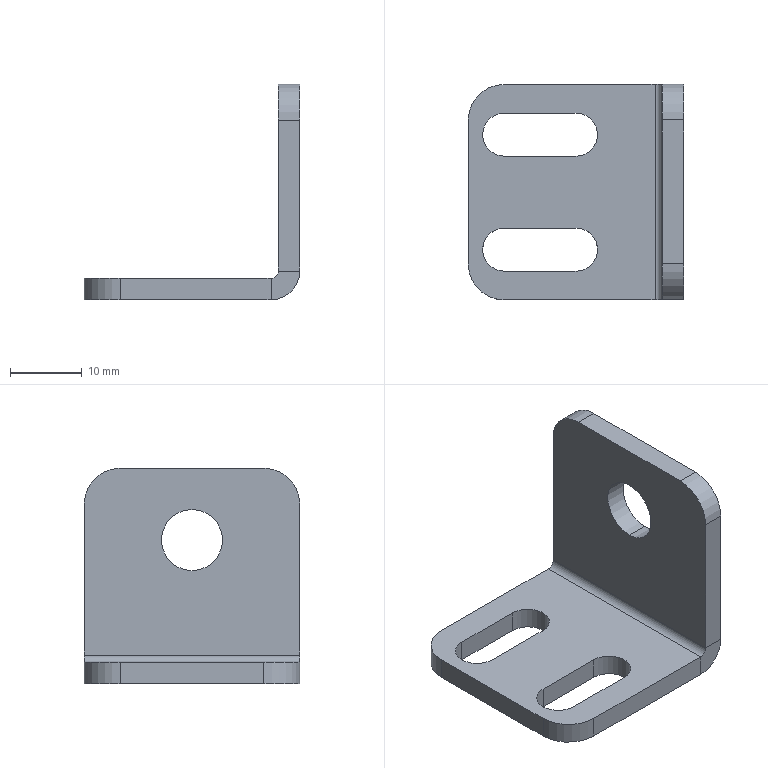Component | SolidWorks | GuideWheelAssembly3-1_RollerBracket1-1 | 1 solid | 28 faces | box 30 x 30 x 30 mm | volume 4269 mm3 | plane 16 | cylinder 12 | commonest cylinder face diameters 6 x4 10 x4 8.5 x2 2 x1 8 x1
STEP:
#1=CARTESIAN_POINT('',(-20.078,-9.252,1.014));
#2=VERTEX_POINT('',#1);
#3=CARTESIAN_POINT('',(-20.078,-9.252,1.348));
#4=VERTEX_POINT('',#3);
#5=CARTESIAN_POINT('',(-20.078,-9.252,1.181));
#6=DIRECTION('',(-1.,-0.,0.));
#7=DIRECTION('',(0.,0.,1.));
#8=AXIS2_PLACEMENT_3D('',#5,#6,#7);
#9=CIRCLE('',#8,0.1673);
#10=EDGE_CURVE('',#2,#4,#9,.T.);
#11=ORIENTED_EDGE('',*,*,#10,.F.);
#12=CARTESIAN_POINT('',(-20.196,-9.252,1.014));
#13=VERTEX_POINT('',#12);
#14=CARTESIAN_POINT('',(-20.078,-9.252,1.014));
#15=DIRECTION('',(-1.,-0.,0.));
#16=VECTOR('',#15,39.37);
#17=LINE('',#14,#16);
#18=EDGE_CURVE('',#2,#13,#17,.T.);
#19=ORIENTED_EDGE('',*,*,#18,.T.);
#20=CARTESIAN_POINT('',(-20.196,-9.252,1.348));
#21=VERTEX_POINT('',#20);
#22=CARTESIAN_POINT('',(-20.196,-9.252,1.181));
#23=DIRECTION('',(-1.,-0.,0.));
#24=DIRECTION('',(0.,0.,1.));
#25=AXIS2_PLACEMENT_3D('',#22,#23,#24);
#26=CIRCLE('',#25,0.1673);
#27=EDGE_CURVE('',#13,#21,#26,.T.);
#28=ORIENTED_EDGE('',*,*,#27,.T.);
#29=CARTESIAN_POINT('',(-20.078,-9.252,1.348));
#30=DIRECTION('',(-1.,-0.,0.));
#31=VECTOR('',#30,39.37);
#32=LINE('',#29,#31);
#33=EDGE_CURVE('',#4,#21,#32,.T.);
#34=ORIENTED_EDGE('',*,*,#33,.F.);
#35=EDGE_LOOP('',(#11,#19,#28,#34));
#36=FACE_OUTER_BOUND('',#35,.T.);
#37=CARTESIAN_POINT('',(-20.078,-9.252,1.181));
#38=DIRECTION('',(-1.,-0.,0.));
#39=DIRECTION('',(0.,0.,1.));
#40=AXIS2_PLACEMENT_3D('',#37,#38,#39);
#41=CYLINDRICAL_SURFACE('',#40,0.1673);
#42=ADVANCED_FACE('',(#36),#41,.F.);
#43=CARTESIAN_POINT('',(-20.078,-8.661,0.5512));
#44=VERTEX_POINT('',#43);
#45=CARTESIAN_POINT('',(-20.196,-8.661,0.5512));
#46=VERTEX_POINT('',#45);
#47=CARTESIAN_POINT('',(-20.078,-8.661,0.5512));
#48=DIRECTION('',(-1.,-0.,0.));
#49=VECTOR('',#48,39.37);
#50=LINE('',#47,#49);
#51=EDGE_CURVE('',#44,#46,#50,.T.);
#52=ORIENTED_EDGE('',*,*,#51,.F.);
#53=CARTESIAN_POINT('',(-20.235,-8.661,0.3937));
#54=VERTEX_POINT('',#53);
#55=CARTESIAN_POINT('',(-20.235,-8.661,0.5512));
#56=DIRECTION('',(-0.,1.,-0.));
#57=DIRECTION('',(1.,0.,0.));
#58=AXIS2_PLACEMENT_3D('',#55,#56,#57);
#59=CIRCLE('',#58,0.1575);
#60=EDGE_CURVE('',#44,#54,#59,.T.);
#61=ORIENTED_EDGE('',*,*,#60,.T.);
#62=CARTESIAN_POINT('',(-20.235,-8.661,0.5118));
#63=VERTEX_POINT('',#62);
#64=CARTESIAN_POINT('',(-20.235,-8.661,0.5118));
#65=DIRECTION('',(-0.,-0.,-1.));
#66=VECTOR('',#65,39.37);
#67=LINE('',#64,#66);
#68=EDGE_CURVE('',#63,#54,#67,.T.);
#69=ORIENTED_EDGE('',*,*,#68,.F.);
#70=CARTESIAN_POINT('',(-20.235,-8.661,0.5512));
#71=DIRECTION('',(-0.,1.,-0.));
#72=DIRECTION('',(-1.,0.,0.));
#73=AXIS2_PLACEMENT_3D('',#70,#71,#72);
#74=CIRCLE('',#73,0.03937);
#75=EDGE_CURVE('',#46,#63,#74,.T.);
#76=ORIENTED_EDGE('',*,*,#75,.F.);
#77=EDGE_LOOP('',(#52,#61,#69,#76));
#78=FACE_OUTER_BOUND('',#77,.T.);
#79=CARTESIAN_POINT('',(-20.078,-8.661,0.5512));
#80=DIRECTION('',(-0.,1.,-0.));
#81=DIRECTION('',(-1.,-0.,0.));
#82=AXIS2_PLACEMENT_3D('',#79,#80,#81);
#83=PLANE('',#82);
#84=ADVANCED_FACE('',(#78),#83,.T.);
#85=CARTESIAN_POINT('',(-20.196,-8.661,1.378));
#86=VERTEX_POINT('',#85);
#87=CARTESIAN_POINT('',(-20.196,-8.661,1.575));
#88=DIRECTION('',(0.,-0.,-1.));
#89=VECTOR('',#88,39.37);
#90=LINE('',#87,#89);
#91=EDGE_CURVE('',#86,#46,#90,.T.);
#92=ORIENTED_EDGE('',*,*,#91,.F.);
#93=CARTESIAN_POINT('',(-20.078,-8.661,1.378));
#94=VERTEX_POINT('',#93);
#95=CARTESIAN_POINT('',(-20.235,-8.661,1.378));
#96=DIRECTION('',(1.,0.,-0.));
#97=VECTOR('',#96,39.37);
#98=LINE('',#95,#97);
#99=EDGE_CURVE('',#86,#94,#98,.T.);
#100=ORIENTED_EDGE('',*,*,#99,.T.);
#101=CARTESIAN_POINT('',(-20.078,-8.661,1.575));
#102=DIRECTION('',(0.,-0.,-1.));
#103=VECTOR('',#102,39.37);
#104=LINE('',#101,#103);
#105=EDGE_CURVE('',#94,#44,#104,.T.);
#106=ORIENTED_EDGE('',*,*,#105,.T.);
#107=ORIENTED_EDGE('',*,*,#51,.T.);
#108=EDGE_LOOP('',(#92,#100,#106,#107));
#109=FACE_OUTER_BOUND('',#108,.T.);
#110=CARTESIAN_POINT('',(-20.235,-8.661,0.5118));
#111=DIRECTION('',(-0.,1.,-0.));
#112=DIRECTION('',(-1.,-0.,0.));
#113=AXIS2_PLACEMENT_3D('',#110,#111,#112);
#114=PLANE('',#113);
#115=ADVANCED_FACE('',(#109),#114,.T.);
#116=CARTESIAN_POINT('',(-20.235,-9.843,0.3937));
#117=VERTEX_POINT('',#116);
#118=CARTESIAN_POINT('',(-20.235,-9.843,0.5118));
#119=VERTEX_POINT('',#118);
#120=CARTESIAN_POINT('',(-20.235,-9.843,0.3937));
#121=DIRECTION('',(0.,0.,1.));
#122=VECTOR('',#121,39.37);
#123=LINE('',#120,#122);
#124=EDGE_CURVE('',#117,#119,#123,.T.);
#125=ORIENTED_EDGE('',*,*,#124,.F.);
#126=CARTESIAN_POINT('',(-20.078,-9.843,0.5512));
#127=VERTEX_POINT('',#126);
#128=CARTESIAN_POINT('',(-20.235,-9.843,0.5512));
#129=DIRECTION('',(-0.,1.,-0.));
#130=DIRECTION('',(1.,0.,0.));
#131=AXIS2_PLACEMENT_3D('',#128,#129,#130);
#132=CIRCLE('',#131,0.1575);
#133=EDGE_CURVE('',#127,#117,#132,.T.);
#134=ORIENTED_EDGE('',*,*,#133,.F.);
#135=CARTESIAN_POINT('',(-20.196,-9.843,0.5512));
#136=VERTEX_POINT('',#135);
#137=CARTESIAN_POINT('',(-20.196,-9.843,0.5512));
#138=DIRECTION('',(1.,0.,-0.));
#139=VECTOR('',#138,39.37);
#140=LINE('',#137,#139);
#141=EDGE_CURVE('',#136,#127,#140,.T.);
#142=ORIENTED_EDGE('',*,*,#141,.F.);
#143=CARTESIAN_POINT('',(-20.235,-9.843,0.5512));
#144=DIRECTION('',(-0.,1.,-0.));
#145=DIRECTION('',(-1.,0.,0.));
#146=AXIS2_PLACEMENT_3D('',#143,#144,#145);
#147=CIRCLE('',#146,0.03937);
#148=EDGE_CURVE('',#136,#119,#147,.T.);
#149=ORIENTED_EDGE('',*,*,#148,.T.);
#150=EDGE_LOOP('',(#125,#134,#142,#149));
#151=FACE_OUTER_BOUND('',#150,.T.);
#152=CARTESIAN_POINT('',(-20.235,-9.843,0.3937));
#153=DIRECTION('',(0.,-1.,0.));
#154=DIRECTION('',(1.,0.,-0.));
#155=AXIS2_PLACEMENT_3D('',#152,#153,#154);
#156=PLANE('',#155);
#157=ADVANCED_FACE('',(#151),#156,.T.);
#158=CARTESIAN_POINT('',(-21.062,-9.843,0.5118));
#159=VERTEX_POINT('',#158);
#160=CARTESIAN_POINT('',(-20.078,-9.843,0.5118));
#161=DIRECTION('',(-1.,-0.,0.));
#162=VECTOR('',#161,39.37);
#163=LINE('',#160,#162);
#164=EDGE_CURVE('',#119,#159,#163,.T.);
#165=ORIENTED_EDGE('',*,*,#164,.T.);
#166=CARTESIAN_POINT('',(-21.062,-9.843,0.3937));
#167=VERTEX_POINT('',#166);
#168=CARTESIAN_POINT('',(-21.062,-9.843,0.5512));
#169=DIRECTION('',(-0.,-0.,-1.));
#170=VECTOR('',#169,39.37);
#171=LINE('',#168,#170);
#172=EDGE_CURVE('',#159,#167,#171,.T.);
#173=ORIENTED_EDGE('',*,*,#172,.T.);
#174=CARTESIAN_POINT('',(-20.078,-9.843,0.3937));
#175=DIRECTION('',(-1.,-0.,0.));
#176=VECTOR('',#175,39.37);
#177=LINE('',#174,#176);
#178=EDGE_CURVE('',#117,#167,#177,.T.);
#179=ORIENTED_EDGE('',*,*,#178,.F.);
#180=ORIENTED_EDGE('',*,*,#124,.T.);
#181=EDGE_LOOP('',(#165,#173,#179,#180));
#182=FACE_OUTER_BOUND('',#181,.T.);
#183=CARTESIAN_POINT('',(-20.196,-9.843,0.5512));
#184=DIRECTION('',(0.,-1.,0.));
#185=DIRECTION('',(1.,0.,-0.));
#186=AXIS2_PLACEMENT_3D('',#183,#184,#185);
#187=PLANE('',#186);
#188=ADVANCED_FACE('',(#182),#187,.T.);
#189=CARTESIAN_POINT('',(-21.062,-9.055,0.3937));
#190=VERTEX_POINT('',#189);
#191=CARTESIAN_POINT('',(-20.668,-9.055,0.3937));
#192=VERTEX_POINT('',#191);
#193=CARTESIAN_POINT('',(-20.668,-9.055,0.3937));
#194=DIRECTION('',(1.,0.,-0.));
#195=VECTOR('',#194,39.37);
#196=LINE('',#193,#195);
#197=EDGE_CURVE('',#190,#192,#196,.T.);
#198=ORIENTED_EDGE('',*,*,#197,.T.);
#199=CARTESIAN_POINT('',(-20.668,-8.819,0.3937));
#200=VERTEX_POINT('',#199);
#201=CARTESIAN_POINT('',(-20.668,-8.937,0.3937));
#202=DIRECTION('',(0.,0.,1.));
#203=DIRECTION('',(0.,-1.,0.));
#204=AXIS2_PLACEMENT_3D('',#201,#202,#203);
#205=CIRCLE('',#204,0.1181);
#206=EDGE_CURVE('',#192,#200,#205,.T.);
#207=ORIENTED_EDGE('',*,*,#206,.T.);
#208=CARTESIAN_POINT('',(-21.062,-8.819,0.3937));
#209=VERTEX_POINT('',#208);
#210=CARTESIAN_POINT('',(-20.668,-8.819,0.3937));
#211=DIRECTION('',(-1.,-0.,0.));
#212=VECTOR('',#211,39.37);
#213=LINE('',#210,#212);
#214=EDGE_CURVE('',#200,#209,#213,.T.);
#215=ORIENTED_EDGE('',*,*,#214,.T.);
#216=CARTESIAN_POINT('',(-21.062,-8.937,0.3937));
#217=DIRECTION('',(0.,0.,1.));
#218=DIRECTION('',(0.,-1.,0.));
#219=AXIS2_PLACEMENT_3D('',#216,#217,#218);
#220=CIRCLE('',#219,0.1181);
#221=EDGE_CURVE('',#209,#190,#220,.T.);
#222=ORIENTED_EDGE('',*,*,#221,.T.);
#223=EDGE_LOOP('',(#198,#207,#215,#222));
#224=FACE_BOUND('',#223,.T.);
#225=CARTESIAN_POINT('',(-21.062,-9.685,0.3937));
#226=VERTEX_POINT('',#225);
#227=CARTESIAN_POINT('',(-20.668,-9.685,0.3937));
#228=VERTEX_POINT('',#227);
#229=CARTESIAN_POINT('',(-20.668,-9.685,0.3937));
#230=DIRECTION('',(1.,0.,-0.));
#231=VECTOR('',#230,39.37);
#232=LINE('',#229,#231);
#233=EDGE_CURVE('',#226,#228,#232,.T.);
#234=ORIENTED_EDGE('',*,*,#233,.T.);
#235=CARTESIAN_POINT('',(-20.668,-9.449,0.3937));
#236=VERTEX_POINT('',#235);
#237=CARTESIAN_POINT('',(-20.668,-9.567,0.3937));
#238=DIRECTION('',(0.,0.,1.));
#239=DIRECTION('',(0.,1.,0.));
#240=AXIS2_PLACEMENT_3D('',#237,#238,#239);
#241=CIRCLE('',#240,0.1181);
#242=EDGE_CURVE('',#228,#236,#241,.T.);
#243=ORIENTED_EDGE('',*,*,#242,.T.);
#244=CARTESIAN_POINT('',(-21.062,-9.449,0.3937));
#245=VERTEX_POINT('',#244);
#246=CARTESIAN_POINT('',(-20.668,-9.449,0.3937));
#247=DIRECTION('',(-1.,-0.,0.));
#248=VECTOR('',#247,39.37);
#249=LINE('',#246,#248);
#250=EDGE_CURVE('',#236,#245,#249,.T.);
#251=ORIENTED_EDGE('',*,*,#250,.T.);
#252=CARTESIAN_POINT('',(-21.062,-9.567,0.3937));
#253=DIRECTION('',(0.,0.,1.));
#254=DIRECTION('',(0.,1.,0.));
#255=AXIS2_PLACEMENT_3D('',#252,#253,#254);
#256=CIRCLE('',#255,0.1181);
#257=EDGE_CURVE('',#245,#226,#256,.T.);
#258=ORIENTED_EDGE('',*,*,#257,.T.);
#259=EDGE_LOOP('',(#234,#243,#251,#258));
#260=FACE_BOUND('',#259,.T.);
#261=CARTESIAN_POINT('',(-21.259,-8.858,0.3937));
#262=VERTEX_POINT('',#261);
#263=CARTESIAN_POINT('',(-21.259,-9.646,0.3937));
#264=VERTEX_POINT('',#263);
#265=CARTESIAN_POINT('',(-21.259,-8.661,0.3937));
#266=DIRECTION('',(0.,-1.,0.));
#267=VECTOR('',#266,39.37);
#268=LINE('',#265,#267);
#269=EDGE_CURVE('',#262,#264,#268,.T.);
#270=ORIENTED_EDGE('',*,*,#269,.F.);
#271=CARTESIAN_POINT('',(-21.062,-8.661,0.3937));
#272=VERTEX_POINT('',#271);
#273=CARTESIAN_POINT('',(-21.062,-8.858,0.3937));
#274=DIRECTION('',(-0.,-0.,-1.));
#275=DIRECTION('',(0.,1.,0.));
#276=AXIS2_PLACEMENT_3D('',#273,#274,#275);
#277=CIRCLE('',#276,0.1969);
#278=EDGE_CURVE('',#262,#272,#277,.T.);
#279=ORIENTED_EDGE('',*,*,#278,.T.);
#280=CARTESIAN_POINT('',(-20.078,-8.661,0.3937));
#281=DIRECTION('',(-1.,-0.,0.));
#282=VECTOR('',#281,39.37);
#283=LINE('',#280,#282);
#284=EDGE_CURVE('',#54,#272,#283,.T.);
#285=ORIENTED_EDGE('',*,*,#284,.F.);
#286=CARTESIAN_POINT('',(-20.235,-8.661,0.3937));
#287=DIRECTION('',(0.,-1.,0.));
#288=VECTOR('',#287,39.37);
#289=LINE('',#286,#288);
#290=EDGE_CURVE('',#54,#117,#289,.T.);
#291=ORIENTED_EDGE('',*,*,#290,.T.);
#292=ORIENTED_EDGE('',*,*,#178,.T.);
#293=CARTESIAN_POINT('',(-21.062,-9.646,0.3937));
#294=DIRECTION('',(-0.,-0.,-1.));
#295=DIRECTION('',(0.,1.,0.));
#296=AXIS2_PLACEMENT_3D('',#293,#294,#295);
#297=CIRCLE('',#296,0.1969);
#298=EDGE_CURVE('',#167,#264,#297,.T.);
#299=ORIENTED_EDGE('',*,*,#298,.T.);
#300=EDGE_LOOP('',(#270,#279,#285,#291,#292,#299));
#301=FACE_OUTER_BOUND('',#300,.T.);
#302=CARTESIAN_POINT('',(-20.078,-8.661,0.3937));
#303=DIRECTION('',(0.,0.,1.));
#304=DIRECTION('',(-0.,1.,-0.));
#305=AXIS2_PLACEMENT_3D('',#302,#303,#304);
#306=PLANE('',#305);
#307=ADVANCED_FACE('',(#224,#260,#301),#306,.F.);
#308=CARTESIAN_POINT('',(-21.259,-8.858,0.5118));
#309=VERTEX_POINT('',#308);
#310=CARTESIAN_POINT('',(-21.259,-9.646,0.5118));
#311=VERTEX_POINT('',#310);
#312=CARTESIAN_POINT('',(-21.259,-8.661,0.5118));
#313=DIRECTION('',(0.,-1.,0.));
#314=VECTOR('',#313,39.37);
#315=LINE('',#312,#314);
#316=EDGE_CURVE('',#309,#311,#315,.T.);
#317=ORIENTED_EDGE('',*,*,#316,.F.);
#318=CARTESIAN_POINT('',(-21.259,-8.858,0.5118));
#319=DIRECTION('',(-0.,-0.,-1.));
#320=VECTOR('',#319,39.37);
#321=LINE('',#318,#320);
#322=EDGE_CURVE('',#309,#262,#321,.T.);
#323=ORIENTED_EDGE('',*,*,#322,.T.);
#324=ORIENTED_EDGE('',*,*,#269,.T.);
#325=CARTESIAN_POINT('',(-21.259,-9.646,0.5118));
#326=DIRECTION('',(0.,0.,1.));
#327=VECTOR('',#326,39.37);
#328=LINE('',#325,#327);
#329=EDGE_CURVE('',#264,#311,#328,.T.);
#330=ORIENTED_EDGE('',*,*,#329,.T.);
#331=EDGE_LOOP('',(#317,#323,#324,#330));
#332=FACE_OUTER_BOUND('',#331,.T.);
#333=CARTESIAN_POINT('',(-21.259,-8.661,0.5118));
#334=DIRECTION('',(-1.,-0.,0.));
#335=DIRECTION('',(0.,-1.,0.));
#336=AXIS2_PLACEMENT_3D('',#333,#334,#335);
#337=PLANE('',#336);
#338=ADVANCED_FACE('',(#332),#337,.T.);
#339=CARTESIAN_POINT('',(-20.668,-9.055,0.5118));
#340=VERTEX_POINT('',#339);
#341=CARTESIAN_POINT('',(-20.668,-8.819,0.5118));
#342=VERTEX_POINT('',#341);
#343=CARTESIAN_POINT('',(-20.668,-8.937,0.5118));
#344=DIRECTION('',(0.,0.,1.));
#345=DIRECTION('',(0.,-1.,0.));
#346=AXIS2_PLACEMENT_3D('',#343,#344,#345);
#347=CIRCLE('',#346,0.1181);
#348=EDGE_CURVE('',#340,#342,#347,.T.);
#349=ORIENTED_EDGE('',*,*,#348,.F.);
#350=CARTESIAN_POINT('',(-21.062,-9.055,0.5118));
#351=VERTEX_POINT('',#350);
#352=CARTESIAN_POINT('',(-20.668,-9.055,0.5118));
#353=DIRECTION('',(1.,0.,-0.));
#354=VECTOR('',#353,39.37);
#355=LINE('',#352,#354);
#356=EDGE_CURVE('',#351,#340,#355,.T.);
#357=ORIENTED_EDGE('',*,*,#356,.F.);
#358=CARTESIAN_POINT('',(-21.062,-8.819,0.5118));
#359=VERTEX_POINT('',#358);
#360=CARTESIAN_POINT('',(-21.062,-8.937,0.5118));
#361=DIRECTION('',(0.,0.,1.));
#362=DIRECTION('',(0.,-1.,0.));
#363=AXIS2_PLACEMENT_3D('',#360,#361,#362);
#364=CIRCLE('',#363,0.1181);
#365=EDGE_CURVE('',#359,#351,#364,.T.);
#366=ORIENTED_EDGE('',*,*,#365,.F.);
#367=CARTESIAN_POINT('',(-20.668,-8.819,0.5118));
#368=DIRECTION('',(-1.,-0.,0.));
#369=VECTOR('',#368,39.37);
#370=LINE('',#367,#369);
#371=EDGE_CURVE('',#342,#359,#370,.T.);
#372=ORIENTED_EDGE('',*,*,#371,.F.);
#373=EDGE_LOOP('',(#349,#357,#366,#372));
#374=FACE_BOUND('',#373,.T.);
#375=CARTESIAN_POINT('',(-20.668,-9.685,0.5118));
#376=VERTEX_POINT('',#375);
#377=CARTESIAN_POINT('',(-20.668,-9.449,0.5118));
#378=VERTEX_POINT('',#377);
#379=CARTESIAN_POINT('',(-20.668,-9.567,0.5118));
#380=DIRECTION('',(0.,0.,1.));
#381=DIRECTION('',(0.,1.,0.));
#382=AXIS2_PLACEMENT_3D('',#379,#380,#381);
#383=CIRCLE('',#382,0.1181);
#384=EDGE_CURVE('',#376,#378,#383,.T.);
#385=ORIENTED_EDGE('',*,*,#384,.F.);
#386=CARTESIAN_POINT('',(-21.062,-9.685,0.5118));
#387=VERTEX_POINT('',#386);
#388=CARTESIAN_POINT('',(-20.668,-9.685,0.5118));
#389=DIRECTION('',(1.,0.,-0.));
#390=VECTOR('',#389,39.37);
#391=LINE('',#388,#390);
#392=EDGE_CURVE('',#387,#376,#391,.T.);
#393=ORIENTED_EDGE('',*,*,#392,.F.);
#394=CARTESIAN_POINT('',(-21.062,-9.449,0.5118));
#395=VERTEX_POINT('',#394);
#396=CARTESIAN_POINT('',(-21.062,-9.567,0.5118));
#397=DIRECTION('',(0.,0.,1.));
#398=DIRECTION('',(0.,1.,0.));
#399=AXIS2_PLACEMENT_3D('',#396,#397,#398);
#400=CIRCLE('',#399,0.1181);
#401=EDGE_CURVE('',#395,#387,#400,.T.);
#402=ORIENTED_EDGE('',*,*,#401,.F.);
#403=CARTESIAN_POINT('',(-20.668,-9.449,0.5118));
#404=DIRECTION('',(-1.,-0.,0.));
#405=VECTOR('',#404,39.37);
#406=LINE('',#403,#405);
#407=EDGE_CURVE('',#378,#395,#406,.T.);
#408=ORIENTED_EDGE('',*,*,#407,.F.);
#409=EDGE_LOOP('',(#385,#393,#402,#408));
#410=FACE_BOUND('',#409,.T.);
#411=CARTESIAN_POINT('',(-21.062,-8.661,0.5118));
#412=VERTEX_POINT('',#411);
#413=CARTESIAN_POINT('',(-20.078,-8.661,0.5118));
#414=DIRECTION('',(-1.,-0.,0.));
#415=VECTOR('',#414,39.37);
#416=LINE('',#413,#415);
#417=EDGE_CURVE('',#63,#412,#416,.T.);
#418=ORIENTED_EDGE('',*,*,#417,.T.);
#419=CARTESIAN_POINT('',(-21.062,-8.858,0.5118));
#420=DIRECTION('',(0.,0.,1.));
#421=DIRECTION('',(0.,1.,0.));
#422=AXIS2_PLACEMENT_3D('',#419,#420,#421);
#423=CIRCLE('',#422,0.1969);
#424=EDGE_CURVE('',#412,#309,#423,.T.);
#425=ORIENTED_EDGE('',*,*,#424,.T.);
#426=ORIENTED_EDGE('',*,*,#316,.T.);
#427=CARTESIAN_POINT('',(-21.062,-9.646,0.5118));
#428=DIRECTION('',(0.,0.,1.));
#429=DIRECTION('',(0.,1.,0.));
#430=AXIS2_PLACEMENT_3D('',#427,#428,#429);
#431=CIRCLE('',#430,0.1969);
#432=EDGE_CURVE('',#311,#159,#431,.T.);
#433=ORIENTED_EDGE('',*,*,#432,.T.);
#434=ORIENTED_EDGE('',*,*,#164,.F.);
#435=CARTESIAN_POINT('',(-20.235,-8.661,0.5118));
#436=DIRECTION('',(0.,-1.,0.));
#437=VECTOR('',#436,39.37);
#438=LINE('',#435,#437);
#439=EDGE_CURVE('',#63,#119,#438,.T.);
#440=ORIENTED_EDGE('',*,*,#439,.F.);
#441=EDGE_LOOP('',(#418,#425,#426,#433,#434,#440));
#442=FACE_OUTER_BOUND('',#441,.T.);
#443=CARTESIAN_POINT('',(-20.078,-8.661,0.5118));
#444=DIRECTION('',(0.,0.,1.));
#445=DIRECTION('',(-0.,1.,-0.));
#446=AXIS2_PLACEMENT_3D('',#443,#444,#445);
#447=PLANE('',#446);
#448=ADVANCED_FACE('',(#374,#410,#442),#447,.T.);
#449=ORIENTED_EDGE('',*,*,#148,.F.);
#450=CARTESIAN_POINT('',(-20.196,-8.661,0.5512));
#451=DIRECTION('',(0.,-1.,0.));
#452=VECTOR('',#451,39.37);
#453=LINE('',#450,#452);
#454=EDGE_CURVE('',#46,#136,#453,.T.);
#455=ORIENTED_EDGE('',*,*,#454,.F.);
#456=ORIENTED_EDGE('',*,*,#75,.T.);
#457=ORIENTED_EDGE('',*,*,#439,.T.);
#458=EDGE_LOOP('',(#449,#455,#456,#457));
#459=FACE_OUTER_BOUND('',#458,.T.);
#460=CARTESIAN_POINT('',(-20.235,-8.661,0.5512));
#461=DIRECTION('',(0.,-1.,0.));
#462=DIRECTION('',(1.,0.,0.));
#463=AXIS2_PLACEMENT_3D('',#460,#461,#462);
#464=CYLINDRICAL_SURFACE('',#463,0.03937);
#465=ADVANCED_FACE('',(#459),#464,.F.);
#466=CARTESIAN_POINT('',(-20.196,-9.252,1.181));
#467=DIRECTION('',(-1.,-0.,0.));
#468=DIRECTION('',(0.,0.,1.));
#469=AXIS2_PLACEMENT_3D('',#466,#467,#468);
#470=CIRCLE('',#469,0.1673);
#471=EDGE_CURVE('',#21,#13,#470,.T.);
#472=ORIENTED_EDGE('',*,*,#471,.F.);
#473=ORIENTED_EDGE('',*,*,#27,.F.);
#474=EDGE_LOOP('',(#472,#473));
#475=FACE_BOUND('',#474,.T.);
#476=CARTESIAN_POINT('',(-20.196,-9.843,1.378));
#477=VERTEX_POINT('',#476);
#478=CARTESIAN_POINT('',(-20.196,-9.843,1.575));
#479=DIRECTION('',(0.,-0.,-1.));
#480=VECTOR('',#479,39.37);
#481=LINE('',#478,#480);
#482=EDGE_CURVE('',#477,#136,#481,.T.);
#483=ORIENTED_EDGE('',*,*,#482,.F.);
#484=CARTESIAN_POINT('',(-20.196,-9.646,1.575));
#485=VERTEX_POINT('',#484);
#486=CARTESIAN_POINT('',(-20.196,-9.646,1.378));
#487=DIRECTION('',(-1.,-0.,-0.));
#488=DIRECTION('',(0.,0.,1.));
#489=AXIS2_PLACEMENT_3D('',#486,#487,#488);
#490=CIRCLE('',#489,0.1969);
#491=EDGE_CURVE('',#477,#485,#490,.T.);
#492=ORIENTED_EDGE('',*,*,#491,.T.);
#493=CARTESIAN_POINT('',(-20.196,-8.858,1.575));
#494=VERTEX_POINT('',#493);
#495=CARTESIAN_POINT('',(-20.196,-8.661,1.575));
#496=DIRECTION('',(0.,-1.,0.));
#497=VECTOR('',#496,39.37);
#498=LINE('',#495,#497);
#499=EDGE_CURVE('',#494,#485,#498,.T.);
#500=ORIENTED_EDGE('',*,*,#499,.F.);
#501=CARTESIAN_POINT('',(-20.196,-8.858,1.378));
#502=DIRECTION('',(-1.,-0.,-0.));
#503=DIRECTION('',(0.,0.,1.));
#504=AXIS2_PLACEMENT_3D('',#501,#502,#503);
#505=CIRCLE('',#504,0.1969);
#506=EDGE_CURVE('',#494,#86,#505,.T.);
#507=ORIENTED_EDGE('',*,*,#506,.T.);
#508=ORIENTED_EDGE('',*,*,#91,.T.);
#509=ORIENTED_EDGE('',*,*,#454,.T.);
#510=EDGE_LOOP('',(#483,#492,#500,#507,#508,#509));
#511=FACE_OUTER_BOUND('',#510,.T.);
#512=CARTESIAN_POINT('',(-20.196,-8.661,1.575));
#513=DIRECTION('',(-1.,-0.,-0.));
#514=DIRECTION('',(-0.,0.,1.));
#515=AXIS2_PLACEMENT_3D('',#512,#513,#514);
#516=PLANE('',#515);
#517=ADVANCED_FACE('',(#475,#511),#516,.T.);
#518=ORIENTED_EDGE('',*,*,#499,.T.);
#519=CARTESIAN_POINT('',(-20.078,-9.646,1.575));
#520=VERTEX_POINT('',#519);
#521=CARTESIAN_POINT('',(-20.078,-9.646,1.575));
#522=DIRECTION('',(1.,0.,-0.));
#523=VECTOR('',#522,39.37);
#524=LINE('',#521,#523);
#525=EDGE_CURVE('',#485,#520,#524,.T.);
#526=ORIENTED_EDGE('',*,*,#525,.T.);
#527=CARTESIAN_POINT('',(-20.078,-8.858,1.575));
#528=VERTEX_POINT('',#527);
#529=CARTESIAN_POINT('',(-20.078,-8.661,1.575));
#530=DIRECTION('',(0.,-1.,0.));
#531=VECTOR('',#530,39.37);
#532=LINE('',#529,#531);
#533=EDGE_CURVE('',#528,#520,#532,.T.);
#534=ORIENTED_EDGE('',*,*,#533,.F.);
#535=CARTESIAN_POINT('',(-20.078,-8.858,1.575));
#536=DIRECTION('',(-1.,-0.,0.));
#537=VECTOR('',#536,39.37);
#538=LINE('',#535,#537);
#539=EDGE_CURVE('',#528,#494,#538,.T.);
#540=ORIENTED_EDGE('',*,*,#539,.T.);
#541=EDGE_LOOP('',(#518,#526,#534,#540));
#542=FACE_OUTER_BOUND('',#541,.T.);
#543=CARTESIAN_POINT('',(-20.078,-8.661,1.575));
#544=DIRECTION('',(0.,0.,1.));
#545=DIRECTION('',(-0.,1.,-0.));
#546=AXIS2_PLACEMENT_3D('',#543,#544,#545);
#547=PLANE('',#546);
#548=ADVANCED_FACE('',(#542),#547,.T.);
#549=CARTESIAN_POINT('',(-20.078,-9.252,1.181));
#550=DIRECTION('',(-1.,-0.,0.));
#551=DIRECTION('',(0.,0.,1.));
#552=AXIS2_PLACEMENT_3D('',#549,#550,#551);
#553=CIRCLE('',#552,0.1673);
#554=EDGE_CURVE('',#4,#2,#553,.T.);
#555=ORIENTED_EDGE('',*,*,#554,.T.);
#556=ORIENTED_EDGE('',*,*,#10,.T.);
#557=EDGE_LOOP('',(#555,#556));
#558=FACE_BOUND('',#557,.T.);
#559=ORIENTED_EDGE('',*,*,#533,.T.);
#560=CARTESIAN_POINT('',(-20.078,-9.843,1.378));
#561=VERTEX_POINT('',#560);
#562=CARTESIAN_POINT('',(-20.078,-9.646,1.378));
#563=DIRECTION('',(1.,0.,0.));
#564=DIRECTION('',(0.,0.,1.));
#565=AXIS2_PLACEMENT_3D('',#562,#563,#564);
#566=CIRCLE('',#565,0.1969);
#567=EDGE_CURVE('',#520,#561,#566,.T.);
#568=ORIENTED_EDGE('',*,*,#567,.T.);
#569=CARTESIAN_POINT('',(-20.078,-9.843,1.575));
#570=DIRECTION('',(0.,-0.,-1.));
#571=VECTOR('',#570,39.37);
#572=LINE('',#569,#571);
#573=EDGE_CURVE('',#561,#127,#572,.T.);
#574=ORIENTED_EDGE('',*,*,#573,.T.);
#575=CARTESIAN_POINT('',(-20.078,-8.661,0.5512));
#576=DIRECTION('',(0.,-1.,0.));
#577=VECTOR('',#576,39.37);
#578=LINE('',#575,#577);
#579=EDGE_CURVE('',#44,#127,#578,.T.);
#580=ORIENTED_EDGE('',*,*,#579,.F.);
#581=ORIENTED_EDGE('',*,*,#105,.F.);
#582=CARTESIAN_POINT('',(-20.078,-8.858,1.378));
#583=DIRECTION('',(1.,0.,0.));
#584=DIRECTION('',(0.,0.,1.));
#585=AXIS2_PLACEMENT_3D('',#582,#583,#584);
#586=CIRCLE('',#585,0.1969);
#587=EDGE_CURVE('',#94,#528,#586,.T.);
#588=ORIENTED_EDGE('',*,*,#587,.T.);
#589=EDGE_LOOP('',(#559,#568,#574,#580,#581,#588));
#590=FACE_OUTER_BOUND('',#589,.T.);
#591=CARTESIAN_POINT('',(-20.078,-8.661,1.575));
#592=DIRECTION('',(-1.,-0.,-0.));
#593=DIRECTION('',(-0.,0.,1.));
#594=AXIS2_PLACEMENT_3D('',#591,#592,#593);
#595=PLANE('',#594);
#596=ADVANCED_FACE('',(#558,#590),#595,.F.);
#597=ORIENTED_EDGE('',*,*,#133,.T.);
#598=ORIENTED_EDGE('',*,*,#290,.F.);
#599=ORIENTED_EDGE('',*,*,#60,.F.);
#600=ORIENTED_EDGE('',*,*,#579,.T.);
#601=EDGE_LOOP('',(#597,#598,#599,#600));
#602=FACE_OUTER_BOUND('',#601,.T.);
#603=CARTESIAN_POINT('',(-20.235,-8.661,0.5512));
#604=DIRECTION('',(0.,-1.,0.));
#605=DIRECTION('',(1.,0.,0.));
#606=AXIS2_PLACEMENT_3D('',#603,#604,#605);
#607=CYLINDRICAL_SURFACE('',#606,0.1575);
#608=ADVANCED_FACE('',(#602),#607,.T.);
#609=ORIENTED_EDGE('',*,*,#284,.T.);
#610=CARTESIAN_POINT('',(-21.062,-8.661,0.5512));
#611=DIRECTION('',(0.,0.,1.));
#612=VECTOR('',#611,39.37);
#613=LINE('',#610,#612);
#614=EDGE_CURVE('',#272,#412,#613,.T.);
#615=ORIENTED_EDGE('',*,*,#614,.T.);
#616=ORIENTED_EDGE('',*,*,#417,.F.);
#617=ORIENTED_EDGE('',*,*,#68,.T.);
#618=EDGE_LOOP('',(#609,#615,#616,#617));
#619=FACE_OUTER_BOUND('',#618,.T.);
#620=CARTESIAN_POINT('',(-20.235,-8.661,0.5512));
#621=DIRECTION('',(-0.,1.,-0.));
#622=DIRECTION('',(-1.,-0.,0.));
#623=AXIS2_PLACEMENT_3D('',#620,#621,#622);
#624=PLANE('',#623);
#625=ADVANCED_FACE('',(#619),#624,.T.);
#626=ORIENTED_EDGE('',*,*,#573,.F.);
#627=CARTESIAN_POINT('',(-20.196,-9.843,1.378));
#628=DIRECTION('',(-1.,-0.,0.));
#629=VECTOR('',#628,39.37);
#630=LINE('',#627,#629);
#631=EDGE_CURVE('',#561,#477,#630,.T.);
#632=ORIENTED_EDGE('',*,*,#631,.T.);
#633=ORIENTED_EDGE('',*,*,#482,.T.);
#634=ORIENTED_EDGE('',*,*,#141,.T.);
#635=EDGE_LOOP('',(#626,#632,#633,#634));
#636=FACE_OUTER_BOUND('',#635,.T.);
#637=CARTESIAN_POINT('',(-20.235,-9.843,0.5512));
#638=DIRECTION('',(-0.,1.,-0.));
#639=DIRECTION('',(-1.,-0.,0.));
#640=AXIS2_PLACEMENT_3D('',#637,#638,#639);
#641=PLANE('',#640);
#642=ADVANCED_FACE('',(#636),#641,.F.);
#643=ORIENTED_EDGE('',*,*,#18,.F.);
#644=ORIENTED_EDGE('',*,*,#554,.F.);
#645=ORIENTED_EDGE('',*,*,#33,.T.);
#646=ORIENTED_EDGE('',*,*,#471,.T.);
#647=EDGE_LOOP('',(#643,#644,#645,#646));
#648=FACE_OUTER_BOUND('',#647,.T.);
#649=CARTESIAN_POINT('',(-20.078,-9.252,1.181));
#650=DIRECTION('',(-1.,-0.,0.));
#651=DIRECTION('',(0.,0.,1.));
#652=AXIS2_PLACEMENT_3D('',#649,#650,#651);
#653=CYLINDRICAL_SURFACE('',#652,0.1673);
#654=ADVANCED_FACE('',(#648),#653,.F.);
#655=ORIENTED_EDGE('',*,*,#384,.T.);
#656=CARTESIAN_POINT('',(-20.668,-9.449,0.3937));
#657=DIRECTION('',(0.,0.,1.));
#658=VECTOR('',#657,39.37);
#659=LINE('',#656,#658);
#660=EDGE_CURVE('',#236,#378,#659,.T.);
#661=ORIENTED_EDGE('',*,*,#660,.F.);
#662=ORIENTED_EDGE('',*,*,#242,.F.);
#663=CARTESIAN_POINT('',(-20.668,-9.685,0.3937));
#664=DIRECTION('',(0.,0.,1.));
#665=VECTOR('',#664,39.37);
#666=LINE('',#663,#665);
#667=EDGE_CURVE('',#228,#376,#666,.T.);
#668=ORIENTED_EDGE('',*,*,#667,.T.);
#669=EDGE_LOOP('',(#655,#661,#662,#668));
#670=FACE_OUTER_BOUND('',#669,.T.);
#671=CARTESIAN_POINT('',(-20.668,-9.567,0.3937));
#672=DIRECTION('',(0.,0.,1.));
#673=DIRECTION('',(0.,1.,0.));
#674=AXIS2_PLACEMENT_3D('',#671,#672,#673);
#675=CYLINDRICAL_SURFACE('',#674,0.1181);
#676=ADVANCED_FACE('',(#670),#675,.F.);
#677=ORIENTED_EDGE('',*,*,#392,.T.);
#678=ORIENTED_EDGE('',*,*,#667,.F.);
#679=ORIENTED_EDGE('',*,*,#233,.F.);
#680=CARTESIAN_POINT('',(-21.062,-9.685,0.3937));
#681=DIRECTION('',(0.,0.,1.));
#682=VECTOR('',#681,39.37);
#683=LINE('',#680,#682);
#684=EDGE_CURVE('',#226,#387,#683,.T.);
#685=ORIENTED_EDGE('',*,*,#684,.T.);
#686=EDGE_LOOP('',(#677,#678,#679,#685));
#687=FACE_OUTER_BOUND('',#686,.T.);
#688=CARTESIAN_POINT('',(-20.668,-9.685,0.3937));
#689=DIRECTION('',(0.,-1.,0.));
#690=DIRECTION('',(1.,0.,-0.));
#691=AXIS2_PLACEMENT_3D('',#688,#689,#690);
#692=PLANE('',#691);
#693=ADVANCED_FACE('',(#687),#692,.F.);
#694=ORIENTED_EDGE('',*,*,#401,.T.);
#695=ORIENTED_EDGE('',*,*,#684,.F.);
#696=ORIENTED_EDGE('',*,*,#257,.F.);
#697=CARTESIAN_POINT('',(-21.062,-9.449,0.3937));
#698=DIRECTION('',(0.,0.,1.));
#699=VECTOR('',#698,39.37);
#700=LINE('',#697,#699);
#701=EDGE_CURVE('',#245,#395,#700,.T.);
#702=ORIENTED_EDGE('',*,*,#701,.T.);
#703=EDGE_LOOP('',(#694,#695,#696,#702));
#704=FACE_OUTER_BOUND('',#703,.T.);
#705=CARTESIAN_POINT('',(-21.062,-9.567,0.3937));
#706=DIRECTION('',(0.,0.,1.));
#707=DIRECTION('',(0.,1.,0.));
#708=AXIS2_PLACEMENT_3D('',#705,#706,#707);
#709=CYLINDRICAL_SURFACE('',#708,0.1181);
#710=ADVANCED_FACE('',(#704),#709,.F.);
#711=ORIENTED_EDGE('',*,*,#407,.T.);
#712=ORIENTED_EDGE('',*,*,#701,.F.);
#713=ORIENTED_EDGE('',*,*,#250,.F.);
#714=ORIENTED_EDGE('',*,*,#660,.T.);
#715=EDGE_LOOP('',(#711,#712,#713,#714));
#716=FACE_OUTER_BOUND('',#715,.T.);
#717=CARTESIAN_POINT('',(-20.668,-9.449,0.3937));
#718=DIRECTION('',(-0.,1.,-0.));
#719=DIRECTION('',(-1.,-0.,0.));
#720=AXIS2_PLACEMENT_3D('',#717,#718,#719);
#721=PLANE('',#720);
#722=ADVANCED_FACE('',(#716),#721,.F.);
#723=ORIENTED_EDGE('',*,*,#348,.T.);
#724=CARTESIAN_POINT('',(-20.668,-8.819,0.3937));
#725=DIRECTION('',(0.,0.,1.));
#726=VECTOR('',#725,39.37);
#727=LINE('',#724,#726);
#728=EDGE_CURVE('',#200,#342,#727,.T.);
#729=ORIENTED_EDGE('',*,*,#728,.F.);
#730=ORIENTED_EDGE('',*,*,#206,.F.);
#731=CARTESIAN_POINT('',(-20.668,-9.055,0.3937));
#732=DIRECTION('',(0.,0.,1.));
#733=VECTOR('',#732,39.37);
#734=LINE('',#731,#733);
#735=EDGE_CURVE('',#192,#340,#734,.T.);
#736=ORIENTED_EDGE('',*,*,#735,.T.);
#737=EDGE_LOOP('',(#723,#729,#730,#736));
#738=FACE_OUTER_BOUND('',#737,.T.);
#739=CARTESIAN_POINT('',(-20.668,-8.937,0.3937));
#740=DIRECTION('',(0.,0.,1.));
#741=DIRECTION('',(0.,1.,0.));
#742=AXIS2_PLACEMENT_3D('',#739,#740,#741);
#743=CYLINDRICAL_SURFACE('',#742,0.1181);
#744=ADVANCED_FACE('',(#738),#743,.F.);
#745=ORIENTED_EDGE('',*,*,#356,.T.);
#746=ORIENTED_EDGE('',*,*,#735,.F.);
#747=ORIENTED_EDGE('',*,*,#197,.F.);
#748=CARTESIAN_POINT('',(-21.062,-9.055,0.3937));
#749=DIRECTION('',(0.,0.,1.));
#750=VECTOR('',#749,39.37);
#751=LINE('',#748,#750);
#752=EDGE_CURVE('',#190,#351,#751,.T.);
#753=ORIENTED_EDGE('',*,*,#752,.T.);
#754=EDGE_LOOP('',(#745,#746,#747,#753));
#755=FACE_OUTER_BOUND('',#754,.T.);
#756=CARTESIAN_POINT('',(-20.668,-9.055,0.3937));
#757=DIRECTION('',(0.,-1.,0.));
#758=DIRECTION('',(1.,0.,-0.));
#759=AXIS2_PLACEMENT_3D('',#756,#757,#758);
#760=PLANE('',#759);
#761=ADVANCED_FACE('',(#755),#760,.F.);
#762=ORIENTED_EDGE('',*,*,#365,.T.);
#763=ORIENTED_EDGE('',*,*,#752,.F.);
#764=ORIENTED_EDGE('',*,*,#221,.F.);
#765=CARTESIAN_POINT('',(-21.062,-8.819,0.3937));
#766=DIRECTION('',(0.,0.,1.));
#767=VECTOR('',#766,39.37);
#768=LINE('',#765,#767);
#769=EDGE_CURVE('',#209,#359,#768,.T.);
#770=ORIENTED_EDGE('',*,*,#769,.T.);
#771=EDGE_LOOP('',(#762,#763,#764,#770));
#772=FACE_OUTER_BOUND('',#771,.T.);
#773=CARTESIAN_POINT('',(-21.062,-8.937,0.3937));
#774=DIRECTION('',(0.,0.,1.));
#775=DIRECTION('',(0.,1.,0.));
#776=AXIS2_PLACEMENT_3D('',#773,#774,#775);
#777=CYLINDRICAL_SURFACE('',#776,0.1181);
#778=ADVANCED_FACE('',(#772),#777,.F.);
#779=ORIENTED_EDGE('',*,*,#371,.T.);
#780=ORIENTED_EDGE('',*,*,#769,.F.);
#781=ORIENTED_EDGE('',*,*,#214,.F.);
#782=ORIENTED_EDGE('',*,*,#728,.T.);
#783=EDGE_LOOP('',(#779,#780,#781,#782));
#784=FACE_OUTER_BOUND('',#783,.T.);
#785=CARTESIAN_POINT('',(-20.668,-8.819,0.3937));
#786=DIRECTION('',(-0.,1.,-0.));
#787=DIRECTION('',(-1.,-0.,0.));
#788=AXIS2_PLACEMENT_3D('',#785,#786,#787);
#789=PLANE('',#788);
#790=ADVANCED_FACE('',(#784),#789,.F.);
#791=ORIENTED_EDGE('',*,*,#424,.F.);
#792=ORIENTED_EDGE('',*,*,#614,.F.);
#793=ORIENTED_EDGE('',*,*,#278,.F.);
#794=ORIENTED_EDGE('',*,*,#322,.F.);
#795=EDGE_LOOP('',(#791,#792,#793,#794));
#796=FACE_OUTER_BOUND('',#795,.T.);
#797=CARTESIAN_POINT('',(-21.062,-8.858,0.5118));
#798=DIRECTION('',(-0.,-0.,-1.));
#799=DIRECTION('',(0.,-1.,0.));
#800=AXIS2_PLACEMENT_3D('',#797,#798,#799);
#801=CYLINDRICAL_SURFACE('',#800,0.1969);
#802=ADVANCED_FACE('',(#796),#801,.T.);
#803=ORIENTED_EDGE('',*,*,#432,.F.);
#804=ORIENTED_EDGE('',*,*,#329,.F.);
#805=ORIENTED_EDGE('',*,*,#298,.F.);
#806=ORIENTED_EDGE('',*,*,#172,.F.);
#807=EDGE_LOOP('',(#803,#804,#805,#806));
#808=FACE_OUTER_BOUND('',#807,.T.);
#809=CARTESIAN_POINT('',(-21.062,-9.646,0.5512));
#810=DIRECTION('',(-0.,-0.,-1.));
#811=DIRECTION('',(0.,-1.,0.));
#812=AXIS2_PLACEMENT_3D('',#809,#810,#811);
#813=CYLINDRICAL_SURFACE('',#812,0.1969);
#814=ADVANCED_FACE('',(#808),#813,.T.);
#815=ORIENTED_EDGE('',*,*,#567,.F.);
#816=ORIENTED_EDGE('',*,*,#525,.F.);
#817=ORIENTED_EDGE('',*,*,#491,.F.);
#818=ORIENTED_EDGE('',*,*,#631,.F.);
#819=EDGE_LOOP('',(#815,#816,#817,#818));
#820=FACE_OUTER_BOUND('',#819,.T.);
#821=CARTESIAN_POINT('',(-20.235,-9.646,1.378));
#822=DIRECTION('',(1.,0.,-0.));
#823=DIRECTION('',(0.,1.,0.));
#824=AXIS2_PLACEMENT_3D('',#821,#822,#823);
#825=CYLINDRICAL_SURFACE('',#824,0.1969);
#826=ADVANCED_FACE('',(#820),#825,.T.);
#827=ORIENTED_EDGE('',*,*,#587,.F.);
#828=ORIENTED_EDGE('',*,*,#99,.F.);
#829=ORIENTED_EDGE('',*,*,#506,.F.);
#830=ORIENTED_EDGE('',*,*,#539,.F.);
#831=EDGE_LOOP('',(#827,#828,#829,#830));
#832=FACE_OUTER_BOUND('',#831,.T.);
#833=CARTESIAN_POINT('',(-20.078,-8.858,1.378));
#834=DIRECTION('',(-1.,-0.,0.));
#835=DIRECTION('',(0.,-1.,0.));
#836=AXIS2_PLACEMENT_3D('',#833,#834,#835);
#837=CYLINDRICAL_SURFACE('',#836,0.1969);
#838=ADVANCED_FACE('',(#832),#837,.T.);
#839=CLOSED_SHELL('',(#42,#84,#115,#157,#188,#307,#338,#448,#465,#517,#548,#596,#608,#625,#642,#654,#676,#693,#710,#722,#744,#761,#778,#790,#802,#814,#826,#838));
#840=MANIFOLD_SOLID_BREP('',#839);
#841=CARTESIAN_POINT('',(0.,0.,0.));
#842=DIRECTION('',(0.,0.,1.));
#843=DIRECTION('',(1.,0.,0.));
#844=AXIS2_PLACEMENT_3D('',#841,#842,#843);
#845=(LENGTH_UNIT()NAMED_UNIT(*)SI_UNIT($,.METRE.));
#846=LENGTH_MEASURE_WITH_UNIT(LENGTH_MEASURE(0.0254),#845);
#847=DIMENSIONAL_EXPONENTS(1.,0.,0.,0.,0.,0.,0.);
#848=(CONVERSION_BASED_UNIT('',#846)LENGTH_UNIT()NAMED_UNIT(#847));
#849=UNCERTAINTY_MEASURE_WITH_UNIT(LENGTH_MEASURE(0.00001),#848,'','');
#850=(NAMED_UNIT(*)PLANE_ANGLE_UNIT()SI_UNIT($,.RADIAN.));
#851=(NAMED_UNIT(*)SI_UNIT($,.STERADIAN.)SOLID_ANGLE_UNIT());
#852=(GEOMETRIC_REPRESENTATION_CONTEXT(3)GLOBAL_UNCERTAINTY_ASSIGNED_CONTEXT((#849))GLOBAL_UNIT_ASSIGNED_CONTEXT((#848,#850,#851))REPRESENTATION_CONTEXT('',''));
#853=ADVANCED_BREP_SHAPE_REPRESENTATION('',(#840,#844),#852);
#854=COLOUR_RGB('',0.7922,0.8196,0.9333);
#855=FILL_AREA_STYLE_COLOUR('',#854);
#856=FILL_AREA_STYLE('',(#855));
#857=SURFACE_STYLE_FILL_AREA(#856);
#858=SURFACE_SIDE_STYLE('',(#857));
#859=SURFACE_STYLE_USAGE(.BOTH.,#858);
#860=PRESENTATION_STYLE_ASSIGNMENT((#859));
#861=STYLED_ITEM('',(#860),#840);
#862=(LENGTH_UNIT()NAMED_UNIT(*)SI_UNIT($,.METRE.));
#863=LENGTH_MEASURE_WITH_UNIT(LENGTH_MEASURE(0.0254),#862);
#864=DIMENSIONAL_EXPONENTS(1.,0.,0.,0.,0.,0.,0.);
#865=(CONVERSION_BASED_UNIT('',#863)LENGTH_UNIT()NAMED_UNIT(#864));
#866=UNCERTAINTY_MEASURE_WITH_UNIT(LENGTH_MEASURE(0.00001),#865,'','');
#867=(NAMED_UNIT(*)PLANE_ANGLE_UNIT()SI_UNIT($,.RADIAN.));
#868=(NAMED_UNIT(*)SI_UNIT($,.STERADIAN.)SOLID_ANGLE_UNIT());
#869=(GEOMETRIC_REPRESENTATION_CONTEXT(3)GLOBAL_UNCERTAINTY_ASSIGNED_CONTEXT((#866))GLOBAL_UNIT_ASSIGNED_CONTEXT((#865,#867,#868))REPRESENTATION_CONTEXT('',''));
#870=MECHANICAL_DESIGN_GEOMETRIC_PRESENTATION_REPRESENTATION('',(#861),#869);
#871=PRESENTATION_LAYER_ASSIGNMENT('','',(#861));